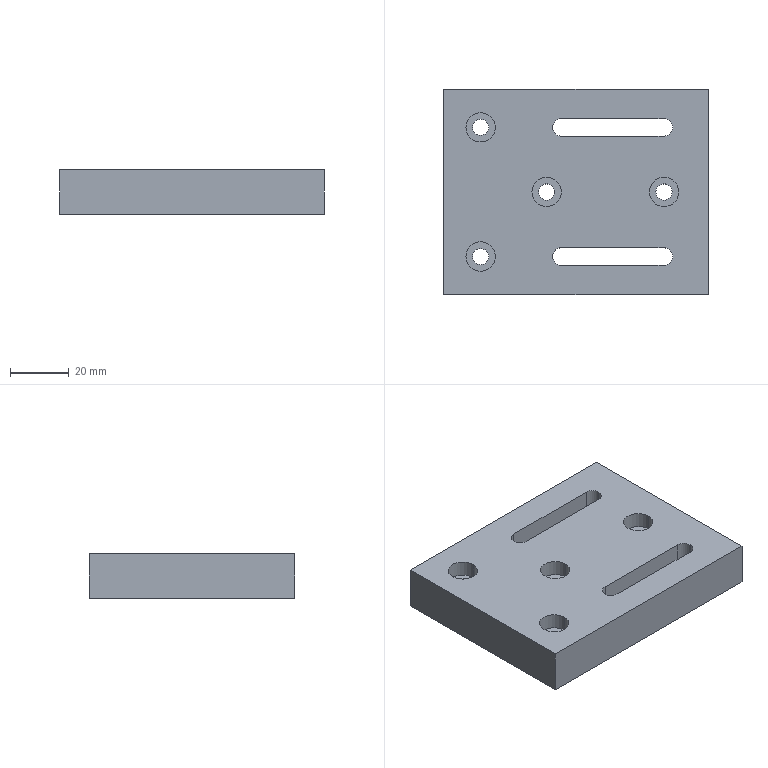Component | SolidWorks | OuterBagSealingBottomPlate-1 | 1 solid | 36 faces | box 90 x 70 x 15 mm | volume 84743 mm3 | cylinder 22 | plane 14 | commonest cylinder face diameters 10 x8 5.5 x8 6 x6
STEP:
#1=COLOUR_RGB('',0.7922,0.8196,0.9333);
#2=FILL_AREA_STYLE_COLOUR('',#1);
#3=FILL_AREA_STYLE('',(#2));
#4=SURFACE_STYLE_FILL_AREA(#3);
#5=SURFACE_SIDE_STYLE('',(#4));
#6=SURFACE_STYLE_USAGE(.BOTH.,#5);
#7=PRESENTATION_STYLE_ASSIGNMENT((#6));
#8=CARTESIAN_POINT('',(2.398,0.5978,2.804));
#9=VERTEX_POINT('',#8);
#10=CARTESIAN_POINT('',(2.28,0.716,2.804));
#11=VERTEX_POINT('',#10);
#12=CARTESIAN_POINT('',(2.28,0.5978,2.804));
#13=DIRECTION('',(0.,0.,1.));
#14=DIRECTION('',(1.,0.,0.));
#15=AXIS2_PLACEMENT_3D('',#12,#13,#14);
#16=CIRCLE('',#15,0.1181);
#17=EDGE_CURVE('',#9,#11,#16,.T.);
#18=ORIENTED_EDGE('',*,*,#17,.F.);
#19=CARTESIAN_POINT('',(2.398,0.5978,3.395));
#20=VERTEX_POINT('',#19);
#21=CARTESIAN_POINT('',(2.398,0.5978,2.804));
#22=DIRECTION('',(0.,0.,1.));
#23=VECTOR('',#22,39.37);
#24=LINE('',#21,#23);
#25=EDGE_CURVE('',#9,#20,#24,.T.);
#26=ORIENTED_EDGE('',*,*,#25,.T.);
#27=CARTESIAN_POINT('',(2.28,0.716,3.395));
#28=VERTEX_POINT('',#27);
#29=CARTESIAN_POINT('',(2.28,0.5978,3.395));
#30=DIRECTION('',(0.,0.,1.));
#31=DIRECTION('',(1.,0.,0.));
#32=AXIS2_PLACEMENT_3D('',#29,#30,#31);
#33=CIRCLE('',#32,0.1181);
#34=EDGE_CURVE('',#20,#28,#33,.T.);
#35=ORIENTED_EDGE('',*,*,#34,.T.);
#36=CARTESIAN_POINT('',(2.28,0.716,2.804));
#37=DIRECTION('',(0.,0.,1.));
#38=VECTOR('',#37,39.37);
#39=LINE('',#36,#38);
#40=EDGE_CURVE('',#11,#28,#39,.T.);
#41=ORIENTED_EDGE('',*,*,#40,.F.);
#42=EDGE_LOOP('',(#18,#26,#35,#41));
#43=FACE_OUTER_BOUND('',#42,.T.);
#44=CARTESIAN_POINT('',(2.28,0.5978,2.804));
#45=DIRECTION('',(0.,0.,1.));
#46=DIRECTION('',(1.,0.,0.));
#47=AXIS2_PLACEMENT_3D('',#44,#45,#46);
#48=CYLINDRICAL_SURFACE('',#47,0.1181);
#49=ADVANCED_FACE('',(#43),#48,.F.);
#50=CARTESIAN_POINT('',(2.398,2.33,2.804));
#51=VERTEX_POINT('',#50);
#52=CARTESIAN_POINT('',(2.28,2.448,2.804));
#53=VERTEX_POINT('',#52);
#54=CARTESIAN_POINT('',(2.28,2.33,2.804));
#55=DIRECTION('',(0.,0.,1.));
#56=DIRECTION('',(1.,0.,0.));
#57=AXIS2_PLACEMENT_3D('',#54,#55,#56);
#58=CIRCLE('',#57,0.1181);
#59=EDGE_CURVE('',#51,#53,#58,.T.);
#60=ORIENTED_EDGE('',*,*,#59,.F.);
#61=CARTESIAN_POINT('',(2.398,2.33,3.395));
#62=VERTEX_POINT('',#61);
#63=CARTESIAN_POINT('',(2.398,2.33,2.804));
#64=DIRECTION('',(0.,0.,1.));
#65=VECTOR('',#64,39.37);
#66=LINE('',#63,#65);
#67=EDGE_CURVE('',#51,#62,#66,.T.);
#68=ORIENTED_EDGE('',*,*,#67,.T.);
#69=CARTESIAN_POINT('',(2.28,2.448,3.395));
#70=VERTEX_POINT('',#69);
#71=CARTESIAN_POINT('',(2.28,2.33,3.395));
#72=DIRECTION('',(0.,0.,1.));
#73=DIRECTION('',(1.,0.,0.));
#74=AXIS2_PLACEMENT_3D('',#71,#72,#73);
#75=CIRCLE('',#74,0.1181);
#76=EDGE_CURVE('',#62,#70,#75,.T.);
#77=ORIENTED_EDGE('',*,*,#76,.T.);
#78=CARTESIAN_POINT('',(2.28,2.448,2.804));
#79=DIRECTION('',(0.,0.,1.));
#80=VECTOR('',#79,39.37);
#81=LINE('',#78,#80);
#82=EDGE_CURVE('',#53,#70,#81,.T.);
#83=ORIENTED_EDGE('',*,*,#82,.F.);
#84=EDGE_LOOP('',(#60,#68,#77,#83));
#85=FACE_OUTER_BOUND('',#84,.T.);
#86=CARTESIAN_POINT('',(2.28,2.33,2.804));
#87=DIRECTION('',(0.,0.,1.));
#88=DIRECTION('',(1.,0.,0.));
#89=AXIS2_PLACEMENT_3D('',#86,#87,#88);
#90=CYLINDRICAL_SURFACE('',#89,0.1181);
#91=ADVANCED_FACE('',(#85),#90,.F.);
#92=CARTESIAN_POINT('',(-0.3773,2.33,3.182));
#93=VERTEX_POINT('',#92);
#94=CARTESIAN_POINT('',(0.01635,2.33,3.182));
#95=VERTEX_POINT('',#94);
#96=CARTESIAN_POINT('',(-0.1805,2.33,3.182));
#97=DIRECTION('',(0.,0.,1.));
#98=DIRECTION('',(1.,0.,0.));
#99=AXIS2_PLACEMENT_3D('',#96,#97,#98);
#100=CIRCLE('',#99,0.1969);
#101=EDGE_CURVE('',#93,#95,#100,.T.);
#102=ORIENTED_EDGE('',*,*,#101,.F.);
#103=CARTESIAN_POINT('',(-0.3773,2.33,3.395));
#104=VERTEX_POINT('',#103);
#105=CARTESIAN_POINT('',(-0.3773,2.33,3.395));
#106=DIRECTION('',(0.,0.,1.));
#107=VECTOR('',#106,39.37);
#108=LINE('',#105,#107);
#109=EDGE_CURVE('',#93,#104,#108,.T.);
#110=ORIENTED_EDGE('',*,*,#109,.T.);
#111=CARTESIAN_POINT('',(0.01635,2.33,3.395));
#112=VERTEX_POINT('',#111);
#113=CARTESIAN_POINT('',(-0.1805,2.33,3.395));
#114=DIRECTION('',(0.,0.,1.));
#115=DIRECTION('',(1.,0.,0.));
#116=AXIS2_PLACEMENT_3D('',#113,#114,#115);
#117=CIRCLE('',#116,0.1969);
#118=EDGE_CURVE('',#104,#112,#117,.T.);
#119=ORIENTED_EDGE('',*,*,#118,.T.);
#120=CARTESIAN_POINT('',(0.01635,2.33,3.395));
#121=DIRECTION('',(0.,0.,1.));
#122=VECTOR('',#121,39.37);
#123=LINE('',#120,#122);
#124=EDGE_CURVE('',#95,#112,#123,.T.);
#125=ORIENTED_EDGE('',*,*,#124,.F.);
#126=EDGE_LOOP('',(#102,#110,#119,#125));
#127=FACE_OUTER_BOUND('',#126,.T.);
#128=CARTESIAN_POINT('',(-0.1805,2.33,3.395));
#129=DIRECTION('',(0.,0.,1.));
#130=DIRECTION('',(1.,0.,0.));
#131=AXIS2_PLACEMENT_3D('',#128,#129,#130);
#132=CYLINDRICAL_SURFACE('',#131,0.1969);
#133=ADVANCED_FACE('',(#127),#132,.F.);
#134=CARTESIAN_POINT('',(-0.2888,2.33,2.804));
#135=VERTEX_POINT('',#134);
#136=CARTESIAN_POINT('',(-0.07223,2.33,2.804));
#137=VERTEX_POINT('',#136);
#138=CARTESIAN_POINT('',(-0.1805,2.33,2.804));
#139=DIRECTION('',(0.,0.,1.));
#140=DIRECTION('',(1.,0.,0.));
#141=AXIS2_PLACEMENT_3D('',#138,#139,#140);
#142=CIRCLE('',#141,0.1083);
#143=EDGE_CURVE('',#135,#137,#142,.T.);
#144=ORIENTED_EDGE('',*,*,#143,.F.);
#145=CARTESIAN_POINT('',(-0.2888,2.33,3.182));
#146=VERTEX_POINT('',#145);
#147=CARTESIAN_POINT('',(-0.2888,2.33,3.395));
#148=DIRECTION('',(0.,0.,1.));
#149=VECTOR('',#148,39.37);
#150=LINE('',#147,#149);
#151=EDGE_CURVE('',#135,#146,#150,.T.);
#152=ORIENTED_EDGE('',*,*,#151,.T.);
#153=CARTESIAN_POINT('',(-0.07223,2.33,3.182));
#154=VERTEX_POINT('',#153);
#155=CARTESIAN_POINT('',(-0.1805,2.33,3.182));
#156=DIRECTION('',(0.,0.,1.));
#157=DIRECTION('',(1.,0.,0.));
#158=AXIS2_PLACEMENT_3D('',#155,#156,#157);
#159=CIRCLE('',#158,0.1083);
#160=EDGE_CURVE('',#146,#154,#159,.T.);
#161=ORIENTED_EDGE('',*,*,#160,.T.);
#162=CARTESIAN_POINT('',(-0.07223,2.33,3.395));
#163=DIRECTION('',(0.,0.,1.));
#164=VECTOR('',#163,39.37);
#165=LINE('',#162,#164);
#166=EDGE_CURVE('',#137,#154,#165,.T.);
#167=ORIENTED_EDGE('',*,*,#166,.F.);
#168=EDGE_LOOP('',(#144,#152,#161,#167));
#169=FACE_OUTER_BOUND('',#168,.T.);
#170=CARTESIAN_POINT('',(-0.1805,2.33,3.395));
#171=DIRECTION('',(0.,0.,1.));
#172=DIRECTION('',(1.,0.,0.));
#173=AXIS2_PLACEMENT_3D('',#170,#171,#172);
#174=CYLINDRICAL_SURFACE('',#173,0.1083);
#175=ADVANCED_FACE('',(#169),#174,.F.);
#176=CARTESIAN_POINT('',(-0.3773,0.5978,3.182));
#177=VERTEX_POINT('',#176);
#178=CARTESIAN_POINT('',(0.01635,0.5978,3.182));
#179=VERTEX_POINT('',#178);
#180=CARTESIAN_POINT('',(-0.1805,0.5978,3.182));
#181=DIRECTION('',(0.,0.,1.));
#182=DIRECTION('',(1.,0.,0.));
#183=AXIS2_PLACEMENT_3D('',#180,#181,#182);
#184=CIRCLE('',#183,0.1969);
#185=EDGE_CURVE('',#177,#179,#184,.T.);
#186=ORIENTED_EDGE('',*,*,#185,.F.);
#187=CARTESIAN_POINT('',(-0.3773,0.5978,3.395));
#188=VERTEX_POINT('',#187);
#189=CARTESIAN_POINT('',(-0.3773,0.5978,3.395));
#190=DIRECTION('',(0.,0.,1.));
#191=VECTOR('',#190,39.37);
#192=LINE('',#189,#191);
#193=EDGE_CURVE('',#177,#188,#192,.T.);
#194=ORIENTED_EDGE('',*,*,#193,.T.);
#195=CARTESIAN_POINT('',(0.01635,0.5978,3.395));
#196=VERTEX_POINT('',#195);
#197=CARTESIAN_POINT('',(-0.1805,0.5978,3.395));
#198=DIRECTION('',(0.,0.,1.));
#199=DIRECTION('',(1.,0.,0.));
#200=AXIS2_PLACEMENT_3D('',#197,#198,#199);
#201=CIRCLE('',#200,0.1969);
#202=EDGE_CURVE('',#188,#196,#201,.T.);
#203=ORIENTED_EDGE('',*,*,#202,.T.);
#204=CARTESIAN_POINT('',(0.01635,0.5978,3.395));
#205=DIRECTION('',(0.,0.,1.));
#206=VECTOR('',#205,39.37);
#207=LINE('',#204,#206);
#208=EDGE_CURVE('',#179,#196,#207,.T.);
#209=ORIENTED_EDGE('',*,*,#208,.F.);
#210=EDGE_LOOP('',(#186,#194,#203,#209));
#211=FACE_OUTER_BOUND('',#210,.T.);
#212=CARTESIAN_POINT('',(-0.1805,0.5978,3.395));
#213=DIRECTION('',(0.,0.,1.));
#214=DIRECTION('',(1.,0.,0.));
#215=AXIS2_PLACEMENT_3D('',#212,#213,#214);
#216=CYLINDRICAL_SURFACE('',#215,0.1969);
#217=ADVANCED_FACE('',(#211),#216,.F.);
#218=CARTESIAN_POINT('',(-0.2888,0.5978,2.804));
#219=VERTEX_POINT('',#218);
#220=CARTESIAN_POINT('',(-0.07223,0.5978,2.804));
#221=VERTEX_POINT('',#220);
#222=CARTESIAN_POINT('',(-0.1805,0.5978,2.804));
#223=DIRECTION('',(0.,0.,1.));
#224=DIRECTION('',(1.,0.,0.));
#225=AXIS2_PLACEMENT_3D('',#222,#223,#224);
#226=CIRCLE('',#225,0.1083);
#227=EDGE_CURVE('',#219,#221,#226,.T.);
#228=ORIENTED_EDGE('',*,*,#227,.F.);
#229=CARTESIAN_POINT('',(-0.2888,0.5978,3.182));
#230=VERTEX_POINT('',#229);
#231=CARTESIAN_POINT('',(-0.2888,0.5978,3.395));
#232=DIRECTION('',(0.,0.,1.));
#233=VECTOR('',#232,39.37);
#234=LINE('',#231,#233);
#235=EDGE_CURVE('',#219,#230,#234,.T.);
#236=ORIENTED_EDGE('',*,*,#235,.T.);
#237=CARTESIAN_POINT('',(-0.07223,0.5978,3.182));
#238=VERTEX_POINT('',#237);
#239=CARTESIAN_POINT('',(-0.1805,0.5978,3.182));
#240=DIRECTION('',(0.,0.,1.));
#241=DIRECTION('',(1.,0.,0.));
#242=AXIS2_PLACEMENT_3D('',#239,#240,#241);
#243=CIRCLE('',#242,0.1083);
#244=EDGE_CURVE('',#230,#238,#243,.T.);
#245=ORIENTED_EDGE('',*,*,#244,.T.);
#246=CARTESIAN_POINT('',(-0.07223,0.5978,3.395));
#247=DIRECTION('',(0.,0.,1.));
#248=VECTOR('',#247,39.37);
#249=LINE('',#246,#248);
#250=EDGE_CURVE('',#221,#238,#249,.T.);
#251=ORIENTED_EDGE('',*,*,#250,.F.);
#252=EDGE_LOOP('',(#228,#236,#245,#251));
#253=FACE_OUTER_BOUND('',#252,.T.);
#254=CARTESIAN_POINT('',(-0.1805,0.5978,3.395));
#255=DIRECTION('',(0.,0.,1.));
#256=DIRECTION('',(1.,0.,0.));
#257=AXIS2_PLACEMENT_3D('',#254,#255,#256);
#258=CYLINDRICAL_SURFACE('',#257,0.1083);
#259=ADVANCED_FACE('',(#253),#258,.F.);
#260=CARTESIAN_POINT('',(0.5085,1.464,3.182));
#261=VERTEX_POINT('',#260);
#262=CARTESIAN_POINT('',(0.9022,1.464,3.182));
#263=VERTEX_POINT('',#262);
#264=CARTESIAN_POINT('',(0.7053,1.464,3.182));
#265=DIRECTION('',(0.,0.,1.));
#266=DIRECTION('',(1.,0.,0.));
#267=AXIS2_PLACEMENT_3D('',#264,#265,#266);
#268=CIRCLE('',#267,0.1969);
#269=EDGE_CURVE('',#261,#263,#268,.T.);
#270=ORIENTED_EDGE('',*,*,#269,.F.);
#271=CARTESIAN_POINT('',(0.5085,1.464,3.395));
#272=VERTEX_POINT('',#271);
#273=CARTESIAN_POINT('',(0.5085,1.464,3.395));
#274=DIRECTION('',(0.,0.,1.));
#275=VECTOR('',#274,39.37);
#276=LINE('',#273,#275);
#277=EDGE_CURVE('',#261,#272,#276,.T.);
#278=ORIENTED_EDGE('',*,*,#277,.T.);
#279=CARTESIAN_POINT('',(0.9022,1.464,3.395));
#280=VERTEX_POINT('',#279);
#281=CARTESIAN_POINT('',(0.7053,1.464,3.395));
#282=DIRECTION('',(0.,0.,1.));
#283=DIRECTION('',(1.,0.,0.));
#284=AXIS2_PLACEMENT_3D('',#281,#282,#283);
#285=CIRCLE('',#284,0.1969);
#286=EDGE_CURVE('',#272,#280,#285,.T.);
#287=ORIENTED_EDGE('',*,*,#286,.T.);
#288=CARTESIAN_POINT('',(0.9022,1.464,3.395));
#289=DIRECTION('',(0.,0.,1.));
#290=VECTOR('',#289,39.37);
#291=LINE('',#288,#290);
#292=EDGE_CURVE('',#263,#280,#291,.T.);
#293=ORIENTED_EDGE('',*,*,#292,.F.);
#294=EDGE_LOOP('',(#270,#278,#287,#293));
#295=FACE_OUTER_BOUND('',#294,.T.);
#296=CARTESIAN_POINT('',(0.7053,1.464,3.395));
#297=DIRECTION('',(0.,0.,1.));
#298=DIRECTION('',(1.,0.,0.));
#299=AXIS2_PLACEMENT_3D('',#296,#297,#298);
#300=CYLINDRICAL_SURFACE('',#299,0.1969);
#301=ADVANCED_FACE('',(#295),#300,.F.);
#302=CARTESIAN_POINT('',(0.5971,1.464,2.804));
#303=VERTEX_POINT('',#302);
#304=CARTESIAN_POINT('',(0.8136,1.464,2.804));
#305=VERTEX_POINT('',#304);
#306=CARTESIAN_POINT('',(0.7053,1.464,2.804));
#307=DIRECTION('',(0.,0.,1.));
#308=DIRECTION('',(1.,0.,0.));
#309=AXIS2_PLACEMENT_3D('',#306,#307,#308);
#310=CIRCLE('',#309,0.1083);
#311=EDGE_CURVE('',#303,#305,#310,.T.);
#312=ORIENTED_EDGE('',*,*,#311,.F.);
#313=CARTESIAN_POINT('',(0.5971,1.464,3.182));
#314=VERTEX_POINT('',#313);
#315=CARTESIAN_POINT('',(0.5971,1.464,3.395));
#316=DIRECTION('',(0.,0.,1.));
#317=VECTOR('',#316,39.37);
#318=LINE('',#315,#317);
#319=EDGE_CURVE('',#303,#314,#318,.T.);
#320=ORIENTED_EDGE('',*,*,#319,.T.);
#321=CARTESIAN_POINT('',(0.8136,1.464,3.182));
#322=VERTEX_POINT('',#321);
#323=CARTESIAN_POINT('',(0.7053,1.464,3.182));
#324=DIRECTION('',(0.,0.,1.));
#325=DIRECTION('',(1.,0.,0.));
#326=AXIS2_PLACEMENT_3D('',#323,#324,#325);
#327=CIRCLE('',#326,0.1083);
#328=EDGE_CURVE('',#314,#322,#327,.T.);
#329=ORIENTED_EDGE('',*,*,#328,.T.);
#330=CARTESIAN_POINT('',(0.8136,1.464,3.395));
#331=DIRECTION('',(0.,0.,1.));
#332=VECTOR('',#331,39.37);
#333=LINE('',#330,#332);
#334=EDGE_CURVE('',#305,#322,#333,.T.);
#335=ORIENTED_EDGE('',*,*,#334,.F.);
#336=EDGE_LOOP('',(#312,#320,#329,#335));
#337=FACE_OUTER_BOUND('',#336,.T.);
#338=CARTESIAN_POINT('',(0.7053,1.464,3.395));
#339=DIRECTION('',(0.,0.,1.));
#340=DIRECTION('',(1.,0.,0.));
#341=AXIS2_PLACEMENT_3D('',#338,#339,#340);
#342=CYLINDRICAL_SURFACE('',#341,0.1083);
#343=ADVANCED_FACE('',(#337),#342,.F.);
#344=CARTESIAN_POINT('',(2.083,1.464,3.182));
#345=VERTEX_POINT('',#344);
#346=CARTESIAN_POINT('',(2.477,1.464,3.182));
#347=VERTEX_POINT('',#346);
#348=CARTESIAN_POINT('',(2.28,1.464,3.182));
#349=DIRECTION('',(0.,0.,1.));
#350=DIRECTION('',(1.,0.,0.));
#351=AXIS2_PLACEMENT_3D('',#348,#349,#350);
#352=CIRCLE('',#351,0.1969);
#353=EDGE_CURVE('',#345,#347,#352,.T.);
#354=ORIENTED_EDGE('',*,*,#353,.F.);
#355=CARTESIAN_POINT('',(2.083,1.464,3.395));
#356=VERTEX_POINT('',#355);
#357=CARTESIAN_POINT('',(2.083,1.464,3.395));
#358=DIRECTION('',(0.,0.,1.));
#359=VECTOR('',#358,39.37);
#360=LINE('',#357,#359);
#361=EDGE_CURVE('',#345,#356,#360,.T.);
#362=ORIENTED_EDGE('',*,*,#361,.T.);
#363=CARTESIAN_POINT('',(2.477,1.464,3.395));
#364=VERTEX_POINT('',#363);
#365=CARTESIAN_POINT('',(2.28,1.464,3.395));
#366=DIRECTION('',(0.,0.,1.));
#367=DIRECTION('',(1.,0.,0.));
#368=AXIS2_PLACEMENT_3D('',#365,#366,#367);
#369=CIRCLE('',#368,0.1969);
#370=EDGE_CURVE('',#356,#364,#369,.T.);
#371=ORIENTED_EDGE('',*,*,#370,.T.);
#372=CARTESIAN_POINT('',(2.477,1.464,3.395));
#373=DIRECTION('',(0.,0.,1.));
#374=VECTOR('',#373,39.37);
#375=LINE('',#372,#374);
#376=EDGE_CURVE('',#347,#364,#375,.T.);
#377=ORIENTED_EDGE('',*,*,#376,.F.);
#378=EDGE_LOOP('',(#354,#362,#371,#377));
#379=FACE_OUTER_BOUND('',#378,.T.);
#380=CARTESIAN_POINT('',(2.28,1.464,3.395));
#381=DIRECTION('',(0.,0.,1.));
#382=DIRECTION('',(1.,0.,0.));
#383=AXIS2_PLACEMENT_3D('',#380,#381,#382);
#384=CYLINDRICAL_SURFACE('',#383,0.1969);
#385=ADVANCED_FACE('',(#379),#384,.F.);
#386=CARTESIAN_POINT('',(2.172,1.464,2.804));
#387=VERTEX_POINT('',#386);
#388=CARTESIAN_POINT('',(2.388,1.464,2.804));
#389=VERTEX_POINT('',#388);
#390=CARTESIAN_POINT('',(2.28,1.464,2.804));
#391=DIRECTION('',(0.,0.,1.));
#392=DIRECTION('',(1.,0.,0.));
#393=AXIS2_PLACEMENT_3D('',#390,#391,#392);
#394=CIRCLE('',#393,0.1083);
#395=EDGE_CURVE('',#387,#389,#394,.T.);
#396=ORIENTED_EDGE('',*,*,#395,.F.);
#397=CARTESIAN_POINT('',(2.172,1.464,3.182));
#398=VERTEX_POINT('',#397);
#399=CARTESIAN_POINT('',(2.172,1.464,3.395));
#400=DIRECTION('',(0.,0.,1.));
#401=VECTOR('',#400,39.37);
#402=LINE('',#399,#401);
#403=EDGE_CURVE('',#387,#398,#402,.T.);
#404=ORIENTED_EDGE('',*,*,#403,.T.);
#405=CARTESIAN_POINT('',(2.388,1.464,3.182));
#406=VERTEX_POINT('',#405);
#407=CARTESIAN_POINT('',(2.28,1.464,3.182));
#408=DIRECTION('',(0.,0.,1.));
#409=DIRECTION('',(1.,0.,0.));
#410=AXIS2_PLACEMENT_3D('',#407,#408,#409);
#411=CIRCLE('',#410,0.1083);
#412=EDGE_CURVE('',#398,#406,#411,.T.);
#413=ORIENTED_EDGE('',*,*,#412,.T.);
#414=CARTESIAN_POINT('',(2.388,1.464,3.395));
#415=DIRECTION('',(0.,0.,1.));
#416=VECTOR('',#415,39.37);
#417=LINE('',#414,#416);
#418=EDGE_CURVE('',#389,#406,#417,.T.);
#419=ORIENTED_EDGE('',*,*,#418,.F.);
#420=EDGE_LOOP('',(#396,#404,#413,#419));
#421=FACE_OUTER_BOUND('',#420,.T.);
#422=CARTESIAN_POINT('',(2.28,1.464,3.395));
#423=DIRECTION('',(0.,0.,1.));
#424=DIRECTION('',(1.,0.,0.));
#425=AXIS2_PLACEMENT_3D('',#422,#423,#424);
#426=CYLINDRICAL_SURFACE('',#425,0.1083);
#427=ADVANCED_FACE('',(#421),#426,.F.);
#428=CARTESIAN_POINT('',(-0.6726,2.842,2.804));
#429=VERTEX_POINT('',#428);
#430=CARTESIAN_POINT('',(-0.6726,0.08603,2.804));
#431=VERTEX_POINT('',#430);
#432=CARTESIAN_POINT('',(-0.6726,0.08603,2.804));
#433=DIRECTION('',(0.,-1.,0.));
#434=VECTOR('',#433,39.37);
#435=LINE('',#432,#434);
#436=EDGE_CURVE('',#429,#431,#435,.T.);
#437=ORIENTED_EDGE('',*,*,#436,.T.);
#438=CARTESIAN_POINT('',(-0.6726,0.08603,3.395));
#439=VERTEX_POINT('',#438);
#440=CARTESIAN_POINT('',(-0.6726,0.08603,3.395));
#441=DIRECTION('',(0.,0.,-1.));
#442=VECTOR('',#441,39.37);
#443=LINE('',#440,#442);
#444=EDGE_CURVE('',#439,#431,#443,.T.);
#445=ORIENTED_EDGE('',*,*,#444,.F.);
#446=CARTESIAN_POINT('',(-0.6726,2.842,3.395));
#447=VERTEX_POINT('',#446);
#448=CARTESIAN_POINT('',(-0.6726,0.08603,3.395));
#449=DIRECTION('',(0.,-1.,0.));
#450=VECTOR('',#449,39.37);
#451=LINE('',#448,#450);
#452=EDGE_CURVE('',#447,#439,#451,.T.);
#453=ORIENTED_EDGE('',*,*,#452,.F.);
#454=CARTESIAN_POINT('',(-0.6726,2.842,3.395));
#455=DIRECTION('',(0.,0.,-1.));
#456=VECTOR('',#455,39.37);
#457=LINE('',#454,#456);
#458=EDGE_CURVE('',#447,#429,#457,.T.);
#459=ORIENTED_EDGE('',*,*,#458,.T.);
#460=EDGE_LOOP('',(#437,#445,#453,#459));
#461=FACE_OUTER_BOUND('',#460,.T.);
#462=CARTESIAN_POINT('',(-0.6726,0.08603,3.395));
#463=DIRECTION('',(1.,0.,0.));
#464=DIRECTION('',(0.,0.,-1.));
#465=AXIS2_PLACEMENT_3D('',#462,#463,#464);
#466=PLANE('',#465);
#467=ADVANCED_FACE('',(#461),#466,.F.);
#468=CARTESIAN_POINT('',(2.871,0.08603,2.804));
#469=VERTEX_POINT('',#468);
#470=CARTESIAN_POINT('',(-0.6726,0.08603,2.804));
#471=DIRECTION('',(1.,0.,0.));
#472=VECTOR('',#471,39.37);
#473=LINE('',#470,#472);
#474=EDGE_CURVE('',#431,#469,#473,.T.);
#475=ORIENTED_EDGE('',*,*,#474,.T.);
#476=CARTESIAN_POINT('',(2.871,0.08603,3.395));
#477=VERTEX_POINT('',#476);
#478=CARTESIAN_POINT('',(2.871,0.08603,3.395));
#479=DIRECTION('',(0.,0.,-1.));
#480=VECTOR('',#479,39.37);
#481=LINE('',#478,#480);
#482=EDGE_CURVE('',#477,#469,#481,.T.);
#483=ORIENTED_EDGE('',*,*,#482,.F.);
#484=CARTESIAN_POINT('',(-0.6726,0.08603,3.395));
#485=DIRECTION('',(1.,0.,0.));
#486=VECTOR('',#485,39.37);
#487=LINE('',#484,#486);
#488=EDGE_CURVE('',#439,#477,#487,.T.);
#489=ORIENTED_EDGE('',*,*,#488,.F.);
#490=ORIENTED_EDGE('',*,*,#444,.T.);
#491=EDGE_LOOP('',(#475,#483,#489,#490));
#492=FACE_OUTER_BOUND('',#491,.T.);
#493=CARTESIAN_POINT('',(-0.6726,0.08603,3.395));
#494=DIRECTION('',(0.,1.,0.));
#495=DIRECTION('',(0.,0.,1.));
#496=AXIS2_PLACEMENT_3D('',#493,#494,#495);
#497=PLANE('',#496);
#498=ADVANCED_FACE('',(#492),#497,.F.);
#499=CARTESIAN_POINT('',(2.871,2.842,2.804));
#500=VERTEX_POINT('',#499);
#501=CARTESIAN_POINT('',(2.871,0.08603,2.804));
#502=DIRECTION('',(0.,1.,0.));
#503=VECTOR('',#502,39.37);
#504=LINE('',#501,#503);
#505=EDGE_CURVE('',#469,#500,#504,.T.);
#506=ORIENTED_EDGE('',*,*,#505,.T.);
#507=CARTESIAN_POINT('',(2.871,2.842,3.395));
#508=VERTEX_POINT('',#507);
#509=CARTESIAN_POINT('',(2.871,2.842,3.395));
#510=DIRECTION('',(0.,0.,-1.));
#511=VECTOR('',#510,39.37);
#512=LINE('',#509,#511);
#513=EDGE_CURVE('',#508,#500,#512,.T.);
#514=ORIENTED_EDGE('',*,*,#513,.F.);
#515=CARTESIAN_POINT('',(2.871,0.08603,3.395));
#516=DIRECTION('',(0.,1.,0.));
#517=VECTOR('',#516,39.37);
#518=LINE('',#515,#517);
#519=EDGE_CURVE('',#477,#508,#518,.T.);
#520=ORIENTED_EDGE('',*,*,#519,.F.);
#521=ORIENTED_EDGE('',*,*,#482,.T.);
#522=EDGE_LOOP('',(#506,#514,#520,#521));
#523=FACE_OUTER_BOUND('',#522,.T.);
#524=CARTESIAN_POINT('',(2.871,0.08603,3.395));
#525=DIRECTION('',(-1.,0.,0.));
#526=DIRECTION('',(0.,0.,1.));
#527=AXIS2_PLACEMENT_3D('',#524,#525,#526);
#528=PLANE('',#527);
#529=ADVANCED_FACE('',(#523),#528,.F.);
#530=CARTESIAN_POINT('',(-0.6726,2.842,2.804));
#531=DIRECTION('',(-1.,0.,0.));
#532=VECTOR('',#531,39.37);
#533=LINE('',#530,#532);
#534=EDGE_CURVE('',#500,#429,#533,.T.);
#535=ORIENTED_EDGE('',*,*,#534,.T.);
#536=ORIENTED_EDGE('',*,*,#458,.F.);
#537=CARTESIAN_POINT('',(-0.6726,2.842,3.395));
#538=DIRECTION('',(-1.,0.,0.));
#539=VECTOR('',#538,39.37);
#540=LINE('',#537,#539);
#541=EDGE_CURVE('',#508,#447,#540,.T.);
#542=ORIENTED_EDGE('',*,*,#541,.F.);
#543=ORIENTED_EDGE('',*,*,#513,.T.);
#544=EDGE_LOOP('',(#535,#536,#542,#543));
#545=FACE_OUTER_BOUND('',#544,.T.);
#546=CARTESIAN_POINT('',(-0.6726,2.842,3.395));
#547=DIRECTION('',(0.,-1.,0.));
#548=DIRECTION('',(0.,0.,-1.));
#549=AXIS2_PLACEMENT_3D('',#546,#547,#548);
#550=PLANE('',#549);
#551=ADVANCED_FACE('',(#545),#550,.F.);
#552=CARTESIAN_POINT('',(0.9022,0.4797,3.395));
#553=VERTEX_POINT('',#552);
#554=CARTESIAN_POINT('',(2.28,0.4797,3.395));
#555=VERTEX_POINT('',#554);
#556=CARTESIAN_POINT('',(0.9022,0.4797,3.395));
#557=DIRECTION('',(1.,0.,0.));
#558=VECTOR('',#557,39.37);
#559=LINE('',#556,#558);
#560=EDGE_CURVE('',#553,#555,#559,.T.);
#561=ORIENTED_EDGE('',*,*,#560,.F.);
#562=CARTESIAN_POINT('',(0.9022,0.716,3.395));
#563=VERTEX_POINT('',#562);
#564=CARTESIAN_POINT('',(0.9022,0.5978,3.395));
#565=DIRECTION('',(0.,0.,1.));
#566=DIRECTION('',(1.,0.,0.));
#567=AXIS2_PLACEMENT_3D('',#564,#565,#566);
#568=CIRCLE('',#567,0.1181);
#569=EDGE_CURVE('',#563,#553,#568,.T.);
#570=ORIENTED_EDGE('',*,*,#569,.F.);
#571=CARTESIAN_POINT('',(0.9022,0.716,3.395));
#572=DIRECTION('',(-1.,0.,0.));
#573=VECTOR('',#572,39.37);
#574=LINE('',#571,#573);
#575=EDGE_CURVE('',#28,#563,#574,.T.);
#576=ORIENTED_EDGE('',*,*,#575,.F.);
#577=ORIENTED_EDGE('',*,*,#34,.F.);
#578=CARTESIAN_POINT('',(2.28,0.5978,3.395));
#579=DIRECTION('',(0.,0.,1.));
#580=DIRECTION('',(1.,0.,0.));
#581=AXIS2_PLACEMENT_3D('',#578,#579,#580);
#582=CIRCLE('',#581,0.1181);
#583=EDGE_CURVE('',#555,#20,#582,.T.);
#584=ORIENTED_EDGE('',*,*,#583,.F.);
#585=EDGE_LOOP('',(#561,#570,#576,#577,#584));
#586=FACE_BOUND('',#585,.T.);
#587=CARTESIAN_POINT('',(0.9022,2.212,3.395));
#588=VERTEX_POINT('',#587);
#589=CARTESIAN_POINT('',(2.28,2.212,3.395));
#590=VERTEX_POINT('',#589);
#591=CARTESIAN_POINT('',(0.9022,2.212,3.395));
#592=DIRECTION('',(1.,0.,0.));
#593=VECTOR('',#592,39.37);
#594=LINE('',#591,#593);
#595=EDGE_CURVE('',#588,#590,#594,.T.);
#596=ORIENTED_EDGE('',*,*,#595,.F.);
#597=CARTESIAN_POINT('',(0.9022,2.448,3.395));
#598=VERTEX_POINT('',#597);
#599=CARTESIAN_POINT('',(0.9022,2.33,3.395));
#600=DIRECTION('',(0.,0.,1.));
#601=DIRECTION('',(1.,0.,0.));
#602=AXIS2_PLACEMENT_3D('',#599,#600,#601);
#603=CIRCLE('',#602,0.1181);
#604=EDGE_CURVE('',#598,#588,#603,.T.);
#605=ORIENTED_EDGE('',*,*,#604,.F.);
#606=CARTESIAN_POINT('',(0.9022,2.448,3.395));
#607=DIRECTION('',(-1.,0.,0.));
#608=VECTOR('',#607,39.37);
#609=LINE('',#606,#608);
#610=EDGE_CURVE('',#70,#598,#609,.T.);
#611=ORIENTED_EDGE('',*,*,#610,.F.);
#612=ORIENTED_EDGE('',*,*,#76,.F.);
#613=CARTESIAN_POINT('',(2.28,2.33,3.395));
#614=DIRECTION('',(0.,0.,1.));
#615=DIRECTION('',(1.,0.,0.));
#616=AXIS2_PLACEMENT_3D('',#613,#614,#615);
#617=CIRCLE('',#616,0.1181);
#618=EDGE_CURVE('',#590,#62,#617,.T.);
#619=ORIENTED_EDGE('',*,*,#618,.F.);
#620=EDGE_LOOP('',(#596,#605,#611,#612,#619));
#621=FACE_BOUND('',#620,.T.);
#622=CARTESIAN_POINT('',(-0.1805,2.33,3.395));
#623=DIRECTION('',(0.,0.,1.));
#624=DIRECTION('',(1.,0.,0.));
#625=AXIS2_PLACEMENT_3D('',#622,#623,#624);
#626=CIRCLE('',#625,0.1969);
#627=EDGE_CURVE('',#112,#104,#626,.T.);
#628=ORIENTED_EDGE('',*,*,#627,.F.);
#629=ORIENTED_EDGE('',*,*,#118,.F.);
#630=EDGE_LOOP('',(#628,#629));
#631=FACE_BOUND('',#630,.T.);
#632=CARTESIAN_POINT('',(-0.1805,0.5978,3.395));
#633=DIRECTION('',(0.,0.,1.));
#634=DIRECTION('',(1.,0.,0.));
#635=AXIS2_PLACEMENT_3D('',#632,#633,#634);
#636=CIRCLE('',#635,0.1969);
#637=EDGE_CURVE('',#196,#188,#636,.T.);
#638=ORIENTED_EDGE('',*,*,#637,.F.);
#639=ORIENTED_EDGE('',*,*,#202,.F.);
#640=EDGE_LOOP('',(#638,#639));
#641=FACE_BOUND('',#640,.T.);
#642=CARTESIAN_POINT('',(0.7053,1.464,3.395));
#643=DIRECTION('',(0.,0.,1.));
#644=DIRECTION('',(1.,0.,0.));
#645=AXIS2_PLACEMENT_3D('',#642,#643,#644);
#646=CIRCLE('',#645,0.1969);
#647=EDGE_CURVE('',#280,#272,#646,.T.);
#648=ORIENTED_EDGE('',*,*,#647,.F.);
#649=ORIENTED_EDGE('',*,*,#286,.F.);
#650=EDGE_LOOP('',(#648,#649));
#651=FACE_BOUND('',#650,.T.);
#652=CARTESIAN_POINT('',(2.28,1.464,3.395));
#653=DIRECTION('',(0.,0.,1.));
#654=DIRECTION('',(1.,0.,0.));
#655=AXIS2_PLACEMENT_3D('',#652,#653,#654);
#656=CIRCLE('',#655,0.1969);
#657=EDGE_CURVE('',#364,#356,#656,.T.);
#658=ORIENTED_EDGE('',*,*,#657,.F.);
#659=ORIENTED_EDGE('',*,*,#370,.F.);
#660=EDGE_LOOP('',(#658,#659));
#661=FACE_BOUND('',#660,.T.);
#662=ORIENTED_EDGE('',*,*,#452,.T.);
#663=ORIENTED_EDGE('',*,*,#488,.T.);
#664=ORIENTED_EDGE('',*,*,#519,.T.);
#665=ORIENTED_EDGE('',*,*,#541,.T.);
#666=EDGE_LOOP('',(#662,#663,#664,#665));
#667=FACE_OUTER_BOUND('',#666,.T.);
#668=CARTESIAN_POINT('',(-0.6726,0.08603,3.395));
#669=DIRECTION('',(0.,0.,-1.));
#670=DIRECTION('',(-1.,0.,0.));
#671=AXIS2_PLACEMENT_3D('',#668,#669,#670);
#672=PLANE('',#671);
#673=ADVANCED_FACE('',(#586,#621,#631,#641,#651,#661,#667),#672,.F.);
#674=CARTESIAN_POINT('',(0.9022,0.716,2.804));
#675=VERTEX_POINT('',#674);
#676=CARTESIAN_POINT('',(0.9022,0.4797,2.804));
#677=VERTEX_POINT('',#676);
#678=CARTESIAN_POINT('',(0.9022,0.5978,2.804));
#679=DIRECTION('',(0.,0.,1.));
#680=DIRECTION('',(1.,0.,0.));
#681=AXIS2_PLACEMENT_3D('',#678,#679,#680);
#682=CIRCLE('',#681,0.1181);
#683=EDGE_CURVE('',#675,#677,#682,.T.);
#684=ORIENTED_EDGE('',*,*,#683,.T.);
#685=CARTESIAN_POINT('',(2.28,0.4797,2.804));
#686=VERTEX_POINT('',#685);
#687=CARTESIAN_POINT('',(0.9022,0.4797,2.804));
#688=DIRECTION('',(1.,0.,0.));
#689=VECTOR('',#688,39.37);
#690=LINE('',#687,#689);
#691=EDGE_CURVE('',#677,#686,#690,.T.);
#692=ORIENTED_EDGE('',*,*,#691,.T.);
#693=CARTESIAN_POINT('',(2.28,0.5978,2.804));
#694=DIRECTION('',(0.,0.,1.));
#695=DIRECTION('',(1.,0.,0.));
#696=AXIS2_PLACEMENT_3D('',#693,#694,#695);
#697=CIRCLE('',#696,0.1181);
#698=EDGE_CURVE('',#686,#9,#697,.T.);
#699=ORIENTED_EDGE('',*,*,#698,.T.);
#700=ORIENTED_EDGE('',*,*,#17,.T.);
#701=CARTESIAN_POINT('',(0.9022,0.716,2.804));
#702=DIRECTION('',(-1.,0.,0.));
#703=VECTOR('',#702,39.37);
#704=LINE('',#701,#703);
#705=EDGE_CURVE('',#11,#675,#704,.T.);
#706=ORIENTED_EDGE('',*,*,#705,.T.);
#707=EDGE_LOOP('',(#684,#692,#699,#700,#706));
#708=FACE_BOUND('',#707,.T.);
#709=CARTESIAN_POINT('',(0.9022,2.448,2.804));
#710=VERTEX_POINT('',#709);
#711=CARTESIAN_POINT('',(0.9022,2.212,2.804));
#712=VERTEX_POINT('',#711);
#713=CARTESIAN_POINT('',(0.9022,2.33,2.804));
#714=DIRECTION('',(0.,0.,1.));
#715=DIRECTION('',(1.,0.,0.));
#716=AXIS2_PLACEMENT_3D('',#713,#714,#715);
#717=CIRCLE('',#716,0.1181);
#718=EDGE_CURVE('',#710,#712,#717,.T.);
#719=ORIENTED_EDGE('',*,*,#718,.T.);
#720=CARTESIAN_POINT('',(2.28,2.212,2.804));
#721=VERTEX_POINT('',#720);
#722=CARTESIAN_POINT('',(0.9022,2.212,2.804));
#723=DIRECTION('',(1.,0.,0.));
#724=VECTOR('',#723,39.37);
#725=LINE('',#722,#724);
#726=EDGE_CURVE('',#712,#721,#725,.T.);
#727=ORIENTED_EDGE('',*,*,#726,.T.);
#728=CARTESIAN_POINT('',(2.28,2.33,2.804));
#729=DIRECTION('',(0.,0.,1.));
#730=DIRECTION('',(1.,0.,0.));
#731=AXIS2_PLACEMENT_3D('',#728,#729,#730);
#732=CIRCLE('',#731,0.1181);
#733=EDGE_CURVE('',#721,#51,#732,.T.);
#734=ORIENTED_EDGE('',*,*,#733,.T.);
#735=ORIENTED_EDGE('',*,*,#59,.T.);
#736=CARTESIAN_POINT('',(0.9022,2.448,2.804));
#737=DIRECTION('',(-1.,0.,0.));
#738=VECTOR('',#737,39.37);
#739=LINE('',#736,#738);
#740=EDGE_CURVE('',#53,#710,#739,.T.);
#741=ORIENTED_EDGE('',*,*,#740,.T.);
#742=EDGE_LOOP('',(#719,#727,#734,#735,#741));
#743=FACE_BOUND('',#742,.T.);
#744=CARTESIAN_POINT('',(-0.1805,2.33,2.804));
#745=DIRECTION('',(0.,0.,1.));
#746=DIRECTION('',(1.,0.,0.));
#747=AXIS2_PLACEMENT_3D('',#744,#745,#746);
#748=CIRCLE('',#747,0.1083);
#749=EDGE_CURVE('',#137,#135,#748,.T.);
#750=ORIENTED_EDGE('',*,*,#749,.T.);
#751=ORIENTED_EDGE('',*,*,#143,.T.);
#752=EDGE_LOOP('',(#750,#751));
#753=FACE_BOUND('',#752,.T.);
#754=CARTESIAN_POINT('',(-0.1805,0.5978,2.804));
#755=DIRECTION('',(0.,0.,1.));
#756=DIRECTION('',(1.,0.,0.));
#757=AXIS2_PLACEMENT_3D('',#754,#755,#756);
#758=CIRCLE('',#757,0.1083);
#759=EDGE_CURVE('',#221,#219,#758,.T.);
#760=ORIENTED_EDGE('',*,*,#759,.T.);
#761=ORIENTED_EDGE('',*,*,#227,.T.);
#762=EDGE_LOOP('',(#760,#761));
#763=FACE_BOUND('',#762,.T.);
#764=CARTESIAN_POINT('',(0.7053,1.464,2.804));
#765=DIRECTION('',(0.,0.,1.));
#766=DIRECTION('',(1.,0.,0.));
#767=AXIS2_PLACEMENT_3D('',#764,#765,#766);
#768=CIRCLE('',#767,0.1083);
#769=EDGE_CURVE('',#305,#303,#768,.T.);
#770=ORIENTED_EDGE('',*,*,#769,.T.);
#771=ORIENTED_EDGE('',*,*,#311,.T.);
#772=EDGE_LOOP('',(#770,#771));
#773=FACE_BOUND('',#772,.T.);
#774=CARTESIAN_POINT('',(2.28,1.464,2.804));
#775=DIRECTION('',(0.,0.,1.));
#776=DIRECTION('',(1.,0.,0.));
#777=AXIS2_PLACEMENT_3D('',#774,#775,#776);
#778=CIRCLE('',#777,0.1083);
#779=EDGE_CURVE('',#389,#387,#778,.T.);
#780=ORIENTED_EDGE('',*,*,#779,.T.);
#781=ORIENTED_EDGE('',*,*,#395,.T.);
#782=EDGE_LOOP('',(#780,#781));
#783=FACE_BOUND('',#782,.T.);
#784=ORIENTED_EDGE('',*,*,#436,.F.);
#785=ORIENTED_EDGE('',*,*,#534,.F.);
#786=ORIENTED_EDGE('',*,*,#505,.F.);
#787=ORIENTED_EDGE('',*,*,#474,.F.);
#788=EDGE_LOOP('',(#784,#785,#786,#787));
#789=FACE_OUTER_BOUND('',#788,.T.);
#790=CARTESIAN_POINT('',(-0.6726,0.08603,2.804));
#791=DIRECTION('',(0.,0.,-1.));
#792=DIRECTION('',(-1.,0.,0.));
#793=AXIS2_PLACEMENT_3D('',#790,#791,#792);
#794=PLANE('',#793);
#795=ADVANCED_FACE('',(#708,#743,#753,#763,#773,#783,#789),#794,.T.);
#796=ORIENTED_EDGE('',*,*,#403,.F.);
#797=ORIENTED_EDGE('',*,*,#779,.F.);
#798=ORIENTED_EDGE('',*,*,#418,.T.);
#799=CARTESIAN_POINT('',(2.28,1.464,3.182));
#800=DIRECTION('',(0.,0.,1.));
#801=DIRECTION('',(1.,0.,0.));
#802=AXIS2_PLACEMENT_3D('',#799,#800,#801);
#803=CIRCLE('',#802,0.1083);
#804=EDGE_CURVE('',#406,#398,#803,.T.);
#805=ORIENTED_EDGE('',*,*,#804,.T.);
#806=EDGE_LOOP('',(#796,#797,#798,#805));
#807=FACE_OUTER_BOUND('',#806,.T.);
#808=CARTESIAN_POINT('',(2.28,1.464,3.395));
#809=DIRECTION('',(0.,0.,1.));
#810=DIRECTION('',(1.,0.,0.));
#811=AXIS2_PLACEMENT_3D('',#808,#809,#810);
#812=CYLINDRICAL_SURFACE('',#811,0.1083);
#813=ADVANCED_FACE('',(#807),#812,.F.);
#814=ORIENTED_EDGE('',*,*,#804,.F.);
#815=ORIENTED_EDGE('',*,*,#412,.F.);
#816=EDGE_LOOP('',(#814,#815));
#817=FACE_BOUND('',#816,.T.);
#818=CARTESIAN_POINT('',(2.28,1.464,3.182));
#819=DIRECTION('',(0.,0.,1.));
#820=DIRECTION('',(1.,0.,0.));
#821=AXIS2_PLACEMENT_3D('',#818,#819,#820);
#822=CIRCLE('',#821,0.1969);
#823=EDGE_CURVE('',#347,#345,#822,.T.);
#824=ORIENTED_EDGE('',*,*,#823,.T.);
#825=ORIENTED_EDGE('',*,*,#353,.T.);
#826=EDGE_LOOP('',(#824,#825));
#827=FACE_OUTER_BOUND('',#826,.T.);
#828=CARTESIAN_POINT('',(2.388,1.464,3.182));
#829=DIRECTION('',(0.,0.,-1.));
#830=DIRECTION('',(-1.,0.,0.));
#831=AXIS2_PLACEMENT_3D('',#828,#829,#830);
#832=PLANE('',#831);
#833=ADVANCED_FACE('',(#817,#827),#832,.F.);
#834=ORIENTED_EDGE('',*,*,#361,.F.);
#835=ORIENTED_EDGE('',*,*,#823,.F.);
#836=ORIENTED_EDGE('',*,*,#376,.T.);
#837=ORIENTED_EDGE('',*,*,#657,.T.);
#838=EDGE_LOOP('',(#834,#835,#836,#837));
#839=FACE_OUTER_BOUND('',#838,.T.);
#840=CARTESIAN_POINT('',(2.28,1.464,3.395));
#841=DIRECTION('',(0.,0.,1.));
#842=DIRECTION('',(1.,0.,0.));
#843=AXIS2_PLACEMENT_3D('',#840,#841,#842);
#844=CYLINDRICAL_SURFACE('',#843,0.1969);
#845=ADVANCED_FACE('',(#839),#844,.F.);
#846=ORIENTED_EDGE('',*,*,#319,.F.);
#847=ORIENTED_EDGE('',*,*,#769,.F.);
#848=ORIENTED_EDGE('',*,*,#334,.T.);
#849=CARTESIAN_POINT('',(0.7053,1.464,3.182));
#850=DIRECTION('',(0.,0.,1.));
#851=DIRECTION('',(1.,0.,0.));
#852=AXIS2_PLACEMENT_3D('',#849,#850,#851);
#853=CIRCLE('',#852,0.1083);
#854=EDGE_CURVE('',#322,#314,#853,.T.);
#855=ORIENTED_EDGE('',*,*,#854,.T.);
#856=EDGE_LOOP('',(#846,#847,#848,#855));
#857=FACE_OUTER_BOUND('',#856,.T.);
#858=CARTESIAN_POINT('',(0.7053,1.464,3.395));
#859=DIRECTION('',(0.,0.,1.));
#860=DIRECTION('',(1.,0.,0.));
#861=AXIS2_PLACEMENT_3D('',#858,#859,#860);
#862=CYLINDRICAL_SURFACE('',#861,0.1083);
#863=ADVANCED_FACE('',(#857),#862,.F.);
#864=ORIENTED_EDGE('',*,*,#854,.F.);
#865=ORIENTED_EDGE('',*,*,#328,.F.);
#866=EDGE_LOOP('',(#864,#865));
#867=FACE_BOUND('',#866,.T.);
#868=CARTESIAN_POINT('',(0.7053,1.464,3.182));
#869=DIRECTION('',(0.,0.,1.));
#870=DIRECTION('',(1.,0.,0.));
#871=AXIS2_PLACEMENT_3D('',#868,#869,#870);
#872=CIRCLE('',#871,0.1969);
#873=EDGE_CURVE('',#263,#261,#872,.T.);
#874=ORIENTED_EDGE('',*,*,#873,.T.);
#875=ORIENTED_EDGE('',*,*,#269,.T.);
#876=EDGE_LOOP('',(#874,#875));
#877=FACE_OUTER_BOUND('',#876,.T.);
#878=CARTESIAN_POINT('',(0.8136,1.464,3.182));
#879=DIRECTION('',(0.,0.,-1.));
#880=DIRECTION('',(-1.,0.,0.));
#881=AXIS2_PLACEMENT_3D('',#878,#879,#880);
#882=PLANE('',#881);
#883=ADVANCED_FACE('',(#867,#877),#882,.F.);
#884=ORIENTED_EDGE('',*,*,#277,.F.);
#885=ORIENTED_EDGE('',*,*,#873,.F.);
#886=ORIENTED_EDGE('',*,*,#292,.T.);
#887=ORIENTED_EDGE('',*,*,#647,.T.);
#888=EDGE_LOOP('',(#884,#885,#886,#887));
#889=FACE_OUTER_BOUND('',#888,.T.);
#890=CARTESIAN_POINT('',(0.7053,1.464,3.395));
#891=DIRECTION('',(0.,0.,1.));
#892=DIRECTION('',(1.,0.,0.));
#893=AXIS2_PLACEMENT_3D('',#890,#891,#892);
#894=CYLINDRICAL_SURFACE('',#893,0.1969);
#895=ADVANCED_FACE('',(#889),#894,.F.);
#896=ORIENTED_EDGE('',*,*,#235,.F.);
#897=ORIENTED_EDGE('',*,*,#759,.F.);
#898=ORIENTED_EDGE('',*,*,#250,.T.);
#899=CARTESIAN_POINT('',(-0.1805,0.5978,3.182));
#900=DIRECTION('',(0.,0.,1.));
#901=DIRECTION('',(1.,0.,0.));
#902=AXIS2_PLACEMENT_3D('',#899,#900,#901);
#903=CIRCLE('',#902,0.1083);
#904=EDGE_CURVE('',#238,#230,#903,.T.);
#905=ORIENTED_EDGE('',*,*,#904,.T.);
#906=EDGE_LOOP('',(#896,#897,#898,#905));
#907=FACE_OUTER_BOUND('',#906,.T.);
#908=CARTESIAN_POINT('',(-0.1805,0.5978,3.395));
#909=DIRECTION('',(0.,0.,1.));
#910=DIRECTION('',(1.,0.,0.));
#911=AXIS2_PLACEMENT_3D('',#908,#909,#910);
#912=CYLINDRICAL_SURFACE('',#911,0.1083);
#913=ADVANCED_FACE('',(#907),#912,.F.);
#914=ORIENTED_EDGE('',*,*,#904,.F.);
#915=ORIENTED_EDGE('',*,*,#244,.F.);
#916=EDGE_LOOP('',(#914,#915));
#917=FACE_BOUND('',#916,.T.);
#918=CARTESIAN_POINT('',(-0.1805,0.5978,3.182));
#919=DIRECTION('',(0.,0.,1.));
#920=DIRECTION('',(1.,0.,0.));
#921=AXIS2_PLACEMENT_3D('',#918,#919,#920);
#922=CIRCLE('',#921,0.1969);
#923=EDGE_CURVE('',#179,#177,#922,.T.);
#924=ORIENTED_EDGE('',*,*,#923,.T.);
#925=ORIENTED_EDGE('',*,*,#185,.T.);
#926=EDGE_LOOP('',(#924,#925));
#927=FACE_OUTER_BOUND('',#926,.T.);
#928=CARTESIAN_POINT('',(-0.07223,0.5978,3.182));
#929=DIRECTION('',(0.,0.,-1.));
#930=DIRECTION('',(-1.,0.,0.));
#931=AXIS2_PLACEMENT_3D('',#928,#929,#930);
#932=PLANE('',#931);
#933=ADVANCED_FACE('',(#917,#927),#932,.F.);
#934=ORIENTED_EDGE('',*,*,#193,.F.);
#935=ORIENTED_EDGE('',*,*,#923,.F.);
#936=ORIENTED_EDGE('',*,*,#208,.T.);
#937=ORIENTED_EDGE('',*,*,#637,.T.);
#938=EDGE_LOOP('',(#934,#935,#936,#937));
#939=FACE_OUTER_BOUND('',#938,.T.);
#940=CARTESIAN_POINT('',(-0.1805,0.5978,3.395));
#941=DIRECTION('',(0.,0.,1.));
#942=DIRECTION('',(1.,0.,0.));
#943=AXIS2_PLACEMENT_3D('',#940,#941,#942);
#944=CYLINDRICAL_SURFACE('',#943,0.1969);
#945=ADVANCED_FACE('',(#939),#944,.F.);
#946=ORIENTED_EDGE('',*,*,#151,.F.);
#947=ORIENTED_EDGE('',*,*,#749,.F.);
#948=ORIENTED_EDGE('',*,*,#166,.T.);
#949=CARTESIAN_POINT('',(-0.1805,2.33,3.182));
#950=DIRECTION('',(0.,0.,1.));
#951=DIRECTION('',(1.,0.,0.));
#952=AXIS2_PLACEMENT_3D('',#949,#950,#951);
#953=CIRCLE('',#952,0.1083);
#954=EDGE_CURVE('',#154,#146,#953,.T.);
#955=ORIENTED_EDGE('',*,*,#954,.T.);
#956=EDGE_LOOP('',(#946,#947,#948,#955));
#957=FACE_OUTER_BOUND('',#956,.T.);
#958=CARTESIAN_POINT('',(-0.1805,2.33,3.395));
#959=DIRECTION('',(0.,0.,1.));
#960=DIRECTION('',(1.,0.,0.));
#961=AXIS2_PLACEMENT_3D('',#958,#959,#960);
#962=CYLINDRICAL_SURFACE('',#961,0.1083);
#963=ADVANCED_FACE('',(#957),#962,.F.);
#964=ORIENTED_EDGE('',*,*,#954,.F.);
#965=ORIENTED_EDGE('',*,*,#160,.F.);
#966=EDGE_LOOP('',(#964,#965));
#967=FACE_BOUND('',#966,.T.);
#968=CARTESIAN_POINT('',(-0.1805,2.33,3.182));
#969=DIRECTION('',(0.,0.,1.));
#970=DIRECTION('',(1.,0.,0.));
#971=AXIS2_PLACEMENT_3D('',#968,#969,#970);
#972=CIRCLE('',#971,0.1969);
#973=EDGE_CURVE('',#95,#93,#972,.T.);
#974=ORIENTED_EDGE('',*,*,#973,.T.);
#975=ORIENTED_EDGE('',*,*,#101,.T.);
#976=EDGE_LOOP('',(#974,#975));
#977=FACE_OUTER_BOUND('',#976,.T.);
#978=CARTESIAN_POINT('',(-0.07223,2.33,3.182));
#979=DIRECTION('',(0.,0.,-1.));
#980=DIRECTION('',(-1.,0.,0.));
#981=AXIS2_PLACEMENT_3D('',#978,#979,#980);
#982=PLANE('',#981);
#983=ADVANCED_FACE('',(#967,#977),#982,.F.);
#984=ORIENTED_EDGE('',*,*,#109,.F.);
#985=ORIENTED_EDGE('',*,*,#973,.F.);
#986=ORIENTED_EDGE('',*,*,#124,.T.);
#987=ORIENTED_EDGE('',*,*,#627,.T.);
#988=EDGE_LOOP('',(#984,#985,#986,#987));
#989=FACE_OUTER_BOUND('',#988,.T.);
#990=CARTESIAN_POINT('',(-0.1805,2.33,3.395));
#991=DIRECTION('',(0.,0.,1.));
#992=DIRECTION('',(1.,0.,0.));
#993=AXIS2_PLACEMENT_3D('',#990,#991,#992);
#994=CYLINDRICAL_SURFACE('',#993,0.1969);
#995=ADVANCED_FACE('',(#989),#994,.F.);
#996=ORIENTED_EDGE('',*,*,#604,.T.);
#997=CARTESIAN_POINT('',(0.9022,2.212,2.804));
#998=DIRECTION('',(0.,0.,1.));
#999=VECTOR('',#998,39.37);
#1000=LINE('',#997,#999);
#1001=EDGE_CURVE('',#712,#588,#1000,.T.);
#1002=ORIENTED_EDGE('',*,*,#1001,.F.);
#1003=ORIENTED_EDGE('',*,*,#718,.F.);
#1004=CARTESIAN_POINT('',(0.9022,2.448,2.804));
#1005=DIRECTION('',(0.,0.,1.));
#1006=VECTOR('',#1005,39.37);
#1007=LINE('',#1004,#1006);
#1008=EDGE_CURVE('',#710,#598,#1007,.T.);
#1009=ORIENTED_EDGE('',*,*,#1008,.T.);
#1010=EDGE_LOOP('',(#996,#1002,#1003,#1009));
#1011=FACE_OUTER_BOUND('',#1010,.T.);
#1012=CARTESIAN_POINT('',(0.9022,2.33,2.804));
#1013=DIRECTION('',(0.,0.,1.));
#1014=DIRECTION('',(1.,0.,0.));
#1015=AXIS2_PLACEMENT_3D('',#1012,#1013,#1014);
#1016=CYLINDRICAL_SURFACE('',#1015,0.1181);
#1017=ADVANCED_FACE('',(#1011),#1016,.F.);
#1018=ORIENTED_EDGE('',*,*,#610,.T.);
#1019=ORIENTED_EDGE('',*,*,#1008,.F.);
#1020=ORIENTED_EDGE('',*,*,#740,.F.);
#1021=ORIENTED_EDGE('',*,*,#82,.T.);
#1022=EDGE_LOOP('',(#1018,#1019,#1020,#1021));
#1023=FACE_OUTER_BOUND('',#1022,.T.);
#1024=CARTESIAN_POINT('',(0.9022,2.448,2.804));
#1025=DIRECTION('',(0.,1.,0.));
#1026=DIRECTION('',(0.,0.,1.));
#1027=AXIS2_PLACEMENT_3D('',#1024,#1025,#1026);
#1028=PLANE('',#1027);
#1029=ADVANCED_FACE('',(#1023),#1028,.F.);
#1030=ORIENTED_EDGE('',*,*,#67,.F.);
#1031=ORIENTED_EDGE('',*,*,#733,.F.);
#1032=CARTESIAN_POINT('',(2.28,2.212,2.804));
#1033=DIRECTION('',(0.,0.,1.));
#1034=VECTOR('',#1033,39.37);
#1035=LINE('',#1032,#1034);
#1036=EDGE_CURVE('',#721,#590,#1035,.T.);
#1037=ORIENTED_EDGE('',*,*,#1036,.T.);
#1038=ORIENTED_EDGE('',*,*,#618,.T.);
#1039=EDGE_LOOP('',(#1030,#1031,#1037,#1038));
#1040=FACE_OUTER_BOUND('',#1039,.T.);
#1041=CARTESIAN_POINT('',(2.28,2.33,2.804));
#1042=DIRECTION('',(0.,0.,1.));
#1043=DIRECTION('',(1.,0.,0.));
#1044=AXIS2_PLACEMENT_3D('',#1041,#1042,#1043);
#1045=CYLINDRICAL_SURFACE('',#1044,0.1181);
#1046=ADVANCED_FACE('',(#1040),#1045,.F.);
#1047=ORIENTED_EDGE('',*,*,#595,.T.);
#1048=ORIENTED_EDGE('',*,*,#1036,.F.);
#1049=ORIENTED_EDGE('',*,*,#726,.F.);
#1050=ORIENTED_EDGE('',*,*,#1001,.T.);
#1051=EDGE_LOOP('',(#1047,#1048,#1049,#1050));
#1052=FACE_OUTER_BOUND('',#1051,.T.);
#1053=CARTESIAN_POINT('',(0.9022,2.212,2.804));
#1054=DIRECTION('',(0.,-1.,0.));
#1055=DIRECTION('',(0.,0.,-1.));
#1056=AXIS2_PLACEMENT_3D('',#1053,#1054,#1055);
#1057=PLANE('',#1056);
#1058=ADVANCED_FACE('',(#1052),#1057,.F.);
#1059=ORIENTED_EDGE('',*,*,#569,.T.);
#1060=CARTESIAN_POINT('',(0.9022,0.4797,2.804));
#1061=DIRECTION('',(0.,0.,1.));
#1062=VECTOR('',#1061,39.37);
#1063=LINE('',#1060,#1062);
#1064=EDGE_CURVE('',#677,#553,#1063,.T.);
#1065=ORIENTED_EDGE('',*,*,#1064,.F.);
#1066=ORIENTED_EDGE('',*,*,#683,.F.);
#1067=CARTESIAN_POINT('',(0.9022,0.716,2.804));
#1068=DIRECTION('',(0.,0.,1.));
#1069=VECTOR('',#1068,39.37);
#1070=LINE('',#1067,#1069);
#1071=EDGE_CURVE('',#675,#563,#1070,.T.);
#1072=ORIENTED_EDGE('',*,*,#1071,.T.);
#1073=EDGE_LOOP('',(#1059,#1065,#1066,#1072));
#1074=FACE_OUTER_BOUND('',#1073,.T.);
#1075=CARTESIAN_POINT('',(0.9022,0.5978,2.804));
#1076=DIRECTION('',(0.,0.,1.));
#1077=DIRECTION('',(1.,0.,0.));
#1078=AXIS2_PLACEMENT_3D('',#1075,#1076,#1077);
#1079=CYLINDRICAL_SURFACE('',#1078,0.1181);
#1080=ADVANCED_FACE('',(#1074),#1079,.F.);
#1081=ORIENTED_EDGE('',*,*,#575,.T.);
#1082=ORIENTED_EDGE('',*,*,#1071,.F.);
#1083=ORIENTED_EDGE('',*,*,#705,.F.);
#1084=ORIENTED_EDGE('',*,*,#40,.T.);
#1085=EDGE_LOOP('',(#1081,#1082,#1083,#1084));
#1086=FACE_OUTER_BOUND('',#1085,.T.);
#1087=CARTESIAN_POINT('',(0.9022,0.716,2.804));
#1088=DIRECTION('',(0.,1.,0.));
#1089=DIRECTION('',(0.,0.,1.));
#1090=AXIS2_PLACEMENT_3D('',#1087,#1088,#1089);
#1091=PLANE('',#1090);
#1092=ADVANCED_FACE('',(#1086),#1091,.F.);
#1093=ORIENTED_EDGE('',*,*,#25,.F.);
#1094=ORIENTED_EDGE('',*,*,#698,.F.);
#1095=CARTESIAN_POINT('',(2.28,0.4797,2.804));
#1096=DIRECTION('',(0.,0.,1.));
#1097=VECTOR('',#1096,39.37);
#1098=LINE('',#1095,#1097);
#1099=EDGE_CURVE('',#686,#555,#1098,.T.);
#1100=ORIENTED_EDGE('',*,*,#1099,.T.);
#1101=ORIENTED_EDGE('',*,*,#583,.T.);
#1102=EDGE_LOOP('',(#1093,#1094,#1100,#1101));
#1103=FACE_OUTER_BOUND('',#1102,.T.);
#1104=CARTESIAN_POINT('',(2.28,0.5978,2.804));
#1105=DIRECTION('',(0.,0.,1.));
#1106=DIRECTION('',(1.,0.,0.));
#1107=AXIS2_PLACEMENT_3D('',#1104,#1105,#1106);
#1108=CYLINDRICAL_SURFACE('',#1107,0.1181);
#1109=ADVANCED_FACE('',(#1103),#1108,.F.);
#1110=ORIENTED_EDGE('',*,*,#560,.T.);
#1111=ORIENTED_EDGE('',*,*,#1099,.F.);
#1112=ORIENTED_EDGE('',*,*,#691,.F.);
#1113=ORIENTED_EDGE('',*,*,#1064,.T.);
#1114=EDGE_LOOP('',(#1110,#1111,#1112,#1113));
#1115=FACE_OUTER_BOUND('',#1114,.T.);
#1116=CARTESIAN_POINT('',(0.9022,0.4797,2.804));
#1117=DIRECTION('',(0.,-1.,0.));
#1118=DIRECTION('',(0.,0.,-1.));
#1119=AXIS2_PLACEMENT_3D('',#1116,#1117,#1118);
#1120=PLANE('',#1119);
#1121=ADVANCED_FACE('',(#1115),#1120,.F.);
#1122=CLOSED_SHELL('',(#49,#91,#133,#175,#217,#259,#301,#343,#385,#427,#467,#498,#529,#551,#673,#795,#813,#833,#845,#863,#883,#895,#913,#933,#945,#963,#983,#995,#1017,#1029,#1046,#1058,#1080,#1092,#1109,#1121));
#1123=MANIFOLD_SOLID_BREP('',#1122);
#1124=STYLED_ITEM('',(#7),#1123);
#1125=PRESENTATION_LAYER_ASSIGNMENT('','',(#1124));
#1126=(LENGTH_UNIT()NAMED_UNIT(*)SI_UNIT($,.METRE.));
#1127=LENGTH_MEASURE_WITH_UNIT(LENGTH_MEASURE(0.0254),#1126);
#1128=DIMENSIONAL_EXPONENTS(1.,0.,0.,0.,0.,0.,0.);
#1129=(CONVERSION_BASED_UNIT('',#1127)LENGTH_UNIT()NAMED_UNIT(#1128));
#1130=UNCERTAINTY_MEASURE_WITH_UNIT(LENGTH_MEASURE(0.00001),#1129,'','');
#1131=(NAMED_UNIT(*)PLANE_ANGLE_UNIT()SI_UNIT($,.RADIAN.));
#1132=(NAMED_UNIT(*)SI_UNIT($,.STERADIAN.)SOLID_ANGLE_UNIT());
#1133=(GEOMETRIC_REPRESENTATION_CONTEXT(3)GLOBAL_UNCERTAINTY_ASSIGNED_CONTEXT((#1130))GLOBAL_UNIT_ASSIGNED_CONTEXT((#1129,#1131,#1132))REPRESENTATION_CONTEXT('',''));
#1134=MECHANICAL_DESIGN_GEOMETRIC_PRESENTATION_REPRESENTATION('',(#1124),#1133);
#1135=CARTESIAN_POINT('',(0.,0.,0.));
#1136=DIRECTION('',(0.,0.,1.));
#1137=DIRECTION('',(1.,0.,0.));
#1138=AXIS2_PLACEMENT_3D('',#1135,#1136,#1137);
#1139=(LENGTH_UNIT()NAMED_UNIT(*)SI_UNIT($,.METRE.));
#1140=LENGTH_MEASURE_WITH_UNIT(LENGTH_MEASURE(0.0254),#1139);
#1141=DIMENSIONAL_EXPONENTS(1.,0.,0.,0.,0.,0.,0.);
#1142=(CONVERSION_BASED_UNIT('',#1140)LENGTH_UNIT()NAMED_UNIT(#1141));
#1143=UNCERTAINTY_MEASURE_WITH_UNIT(LENGTH_MEASURE(0.00001),#1142,'','');
#1144=(NAMED_UNIT(*)PLANE_ANGLE_UNIT()SI_UNIT($,.RADIAN.));
#1145=(NAMED_UNIT(*)SI_UNIT($,.STERADIAN.)SOLID_ANGLE_UNIT());
#1146=(GEOMETRIC_REPRESENTATION_CONTEXT(3)GLOBAL_UNCERTAINTY_ASSIGNED_CONTEXT((#1143))GLOBAL_UNIT_ASSIGNED_CONTEXT((#1142,#1144,#1145))REPRESENTATION_CONTEXT('',''));
#1147=ADVANCED_BREP_SHAPE_REPRESENTATION('',(#1123,#1138),#1146);